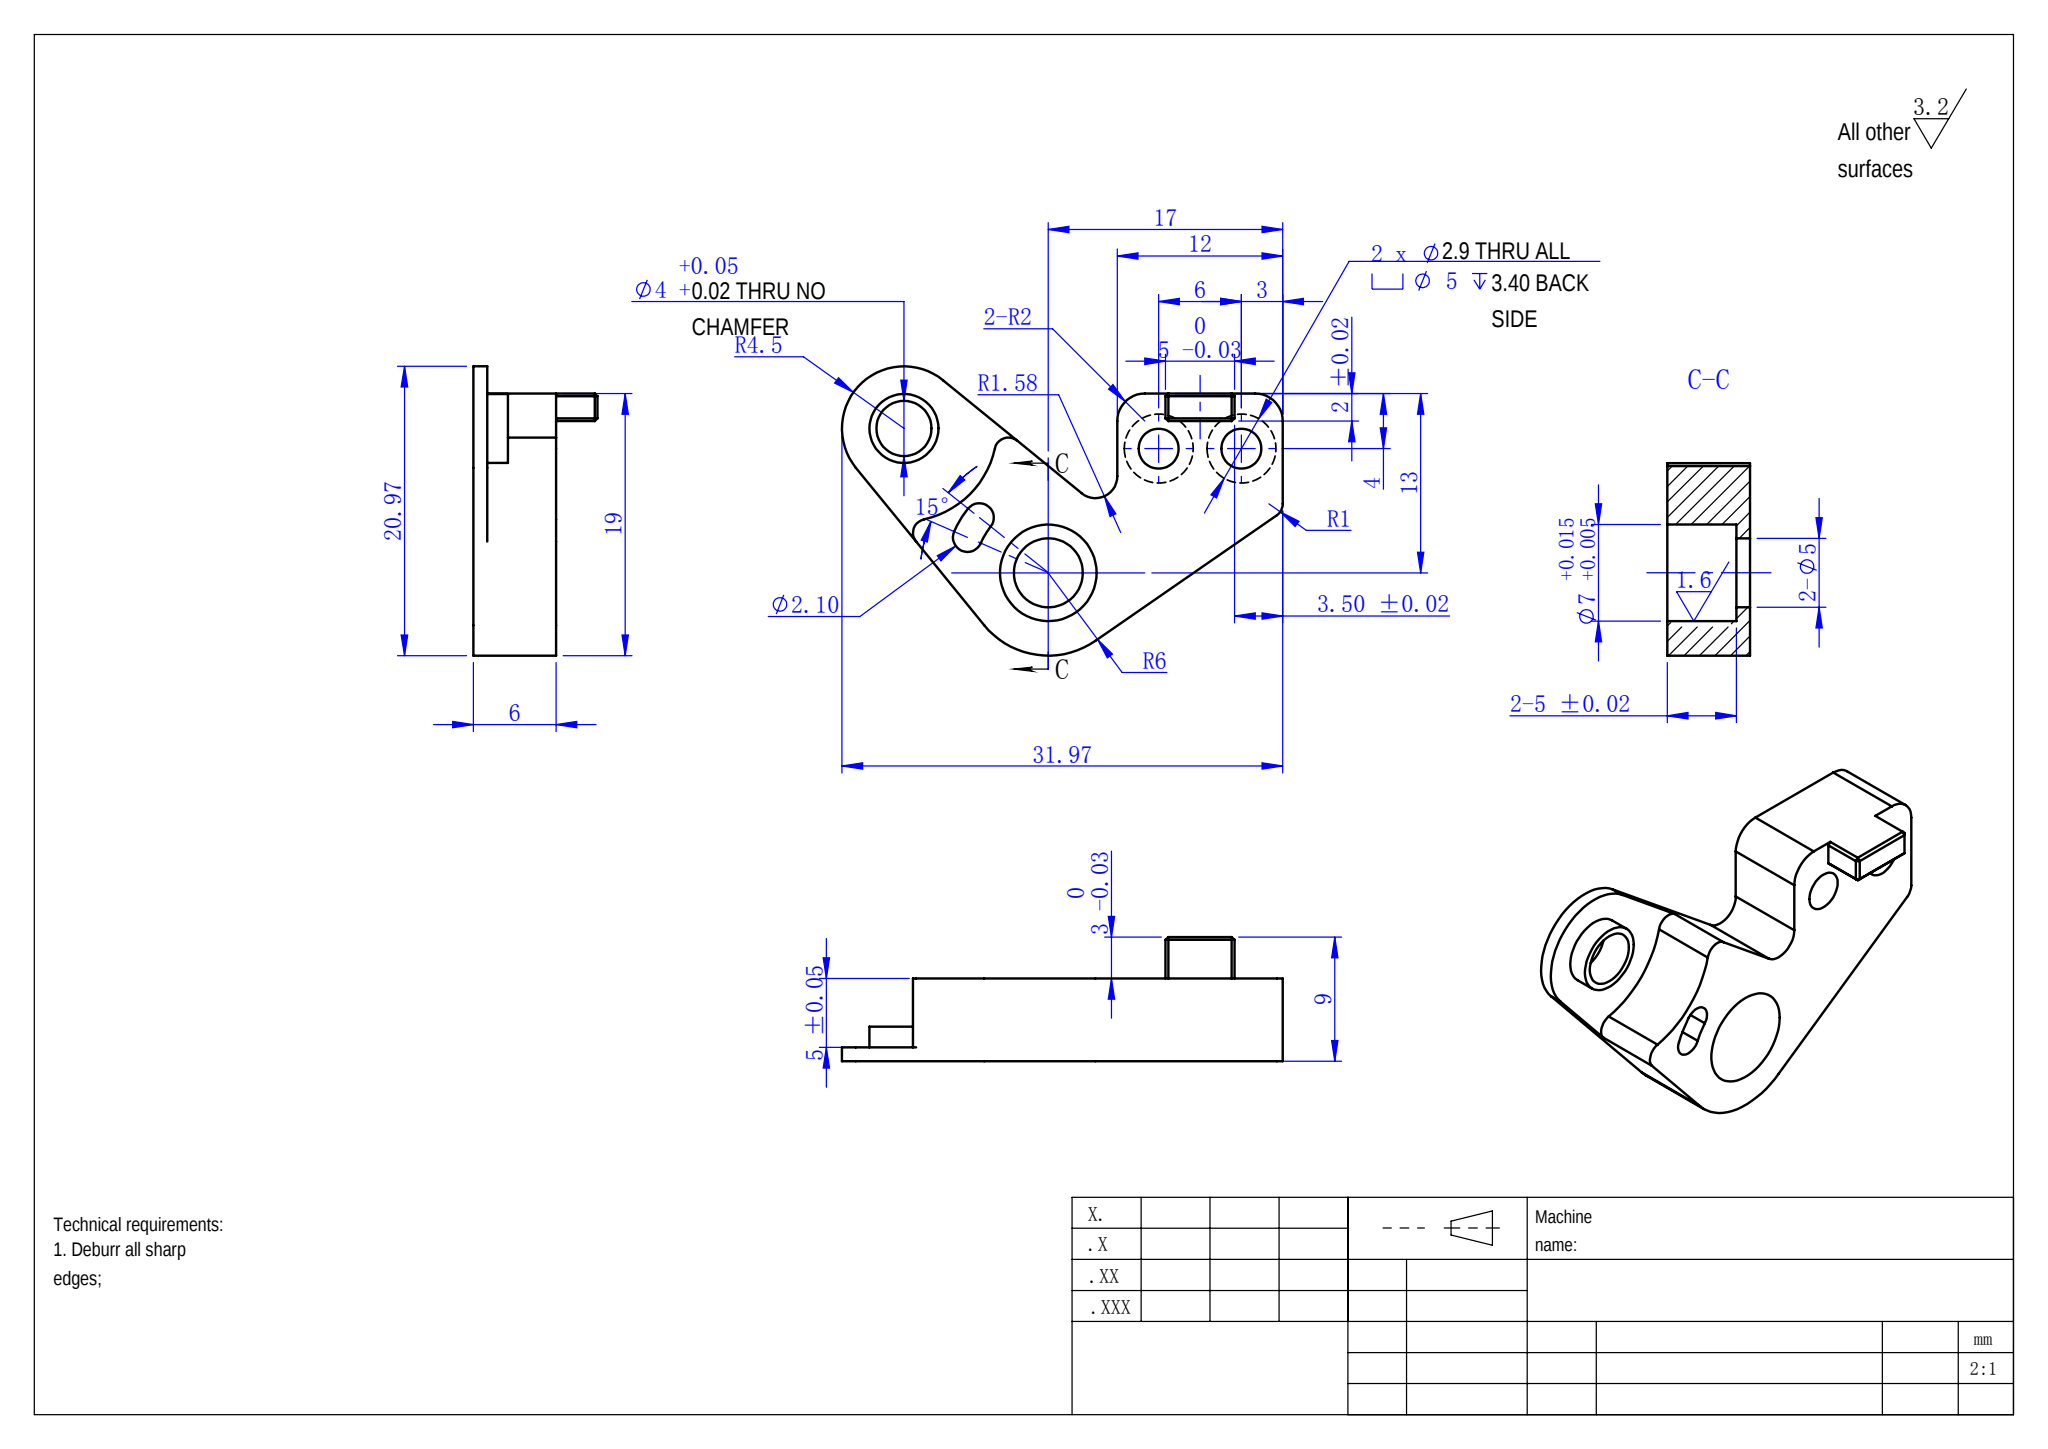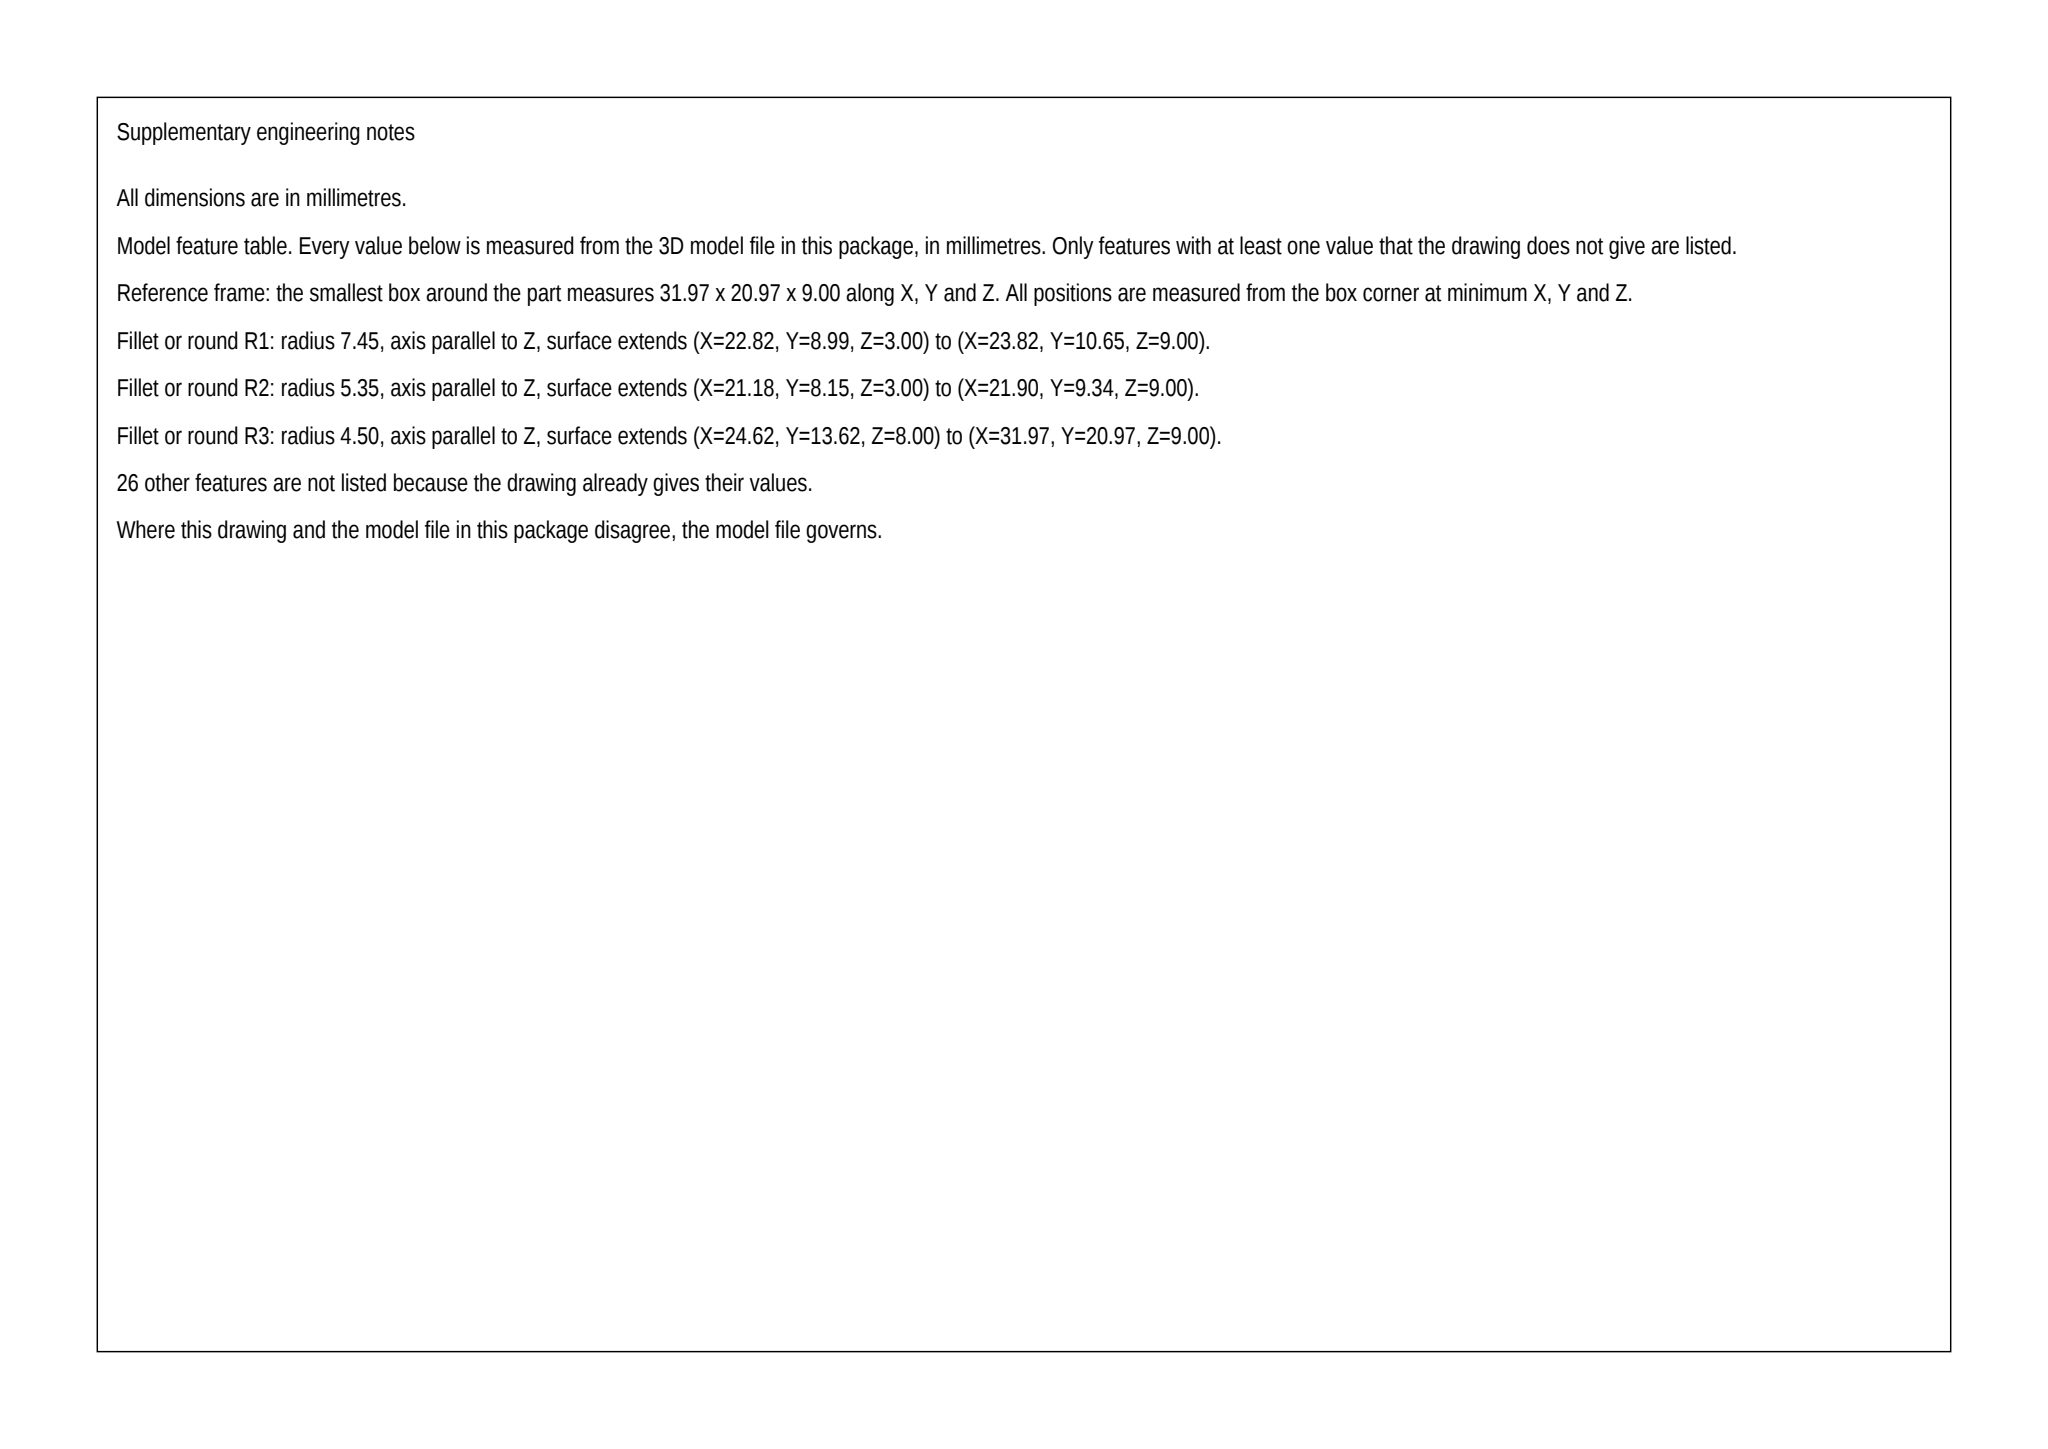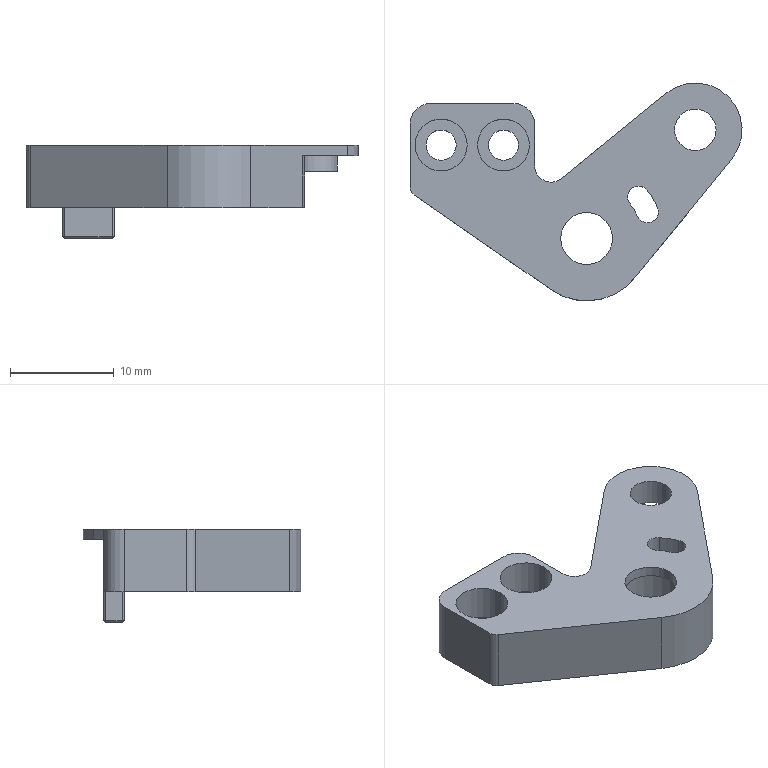Part | SolidWorks | mm | 1 solid | 59 faces | box 31.97 x 20.97 x 9 mm | volume 1507 mm3 | cylinder 30 | plane 29 | commonest cylinder face diameters 5 x8 2.9 x4 4 x4 2.1 x3 2 x3 7 x2 3.168 x1 12 x1
Drawing notes:
R1.58 notch radius centre located at X13.58/Y13.00 from the lower-left corner. | from the solid: cylinder dia 3.168 (=R1.584), axis z, pos (13.58,13.0), length 6.0
R1 half-round notch on right-hand edge: centre at X25.81/Y8.89 from the lower-left corner, 5 deep; second R1 notch centre at X19.89/Y14.81. | from the solid: cylinders dia 2.0, axis z, pos (25.81,8.89) and (19.89,14.81), length 5.0
Ø7 +0.015/+0.005 bore / R6 boss centre located at X17.00/Y6.00 from the lower-left corner. | from the solid: cylinders dia 7.0, 10.7, 12.0, 14.9, axis z, pos (17.0,6.0)
2X Ø2.9 DP 2.6 FROM NEAR FACE, CBORE Ø5 DP 3.4 FROM FAR SIDE (THRU 6 PLATE); CENTRES X3.0 Y15.0 AND X9.0 Y15.0 FROM LOWER-LEFT CORNER DATUM | from the solid: cylinders dia 2.9 len 2.6 and dia 5.0 len 3.4, both axis z at [3.0,15.0] and [9.0,15.0]
COUNTERBORED HOLE ON UPPER ARM: Ø4 DP 2.5 (Z6.5 TO Z9.0), CBORE Ø5 DP 1.5 (Z6.5 TO Z8.0), BOSS Ø9 DP 1.0 (Z8.0 TO Z9.0) ON Ø13.5; CENTRE X27.5 Y16.5 FROM LOWER-LEFT CORNER DATUM | from the solid: hole/bore Ø4 z @ [27.5,16.5] from 6.5 to 9.0; boss/shaft Ø5 @ [27.5,16.5] from 6.5 to 8.0; convex arc Ø9 @ [27.5,16.5] from 8.0 to 9.0; concave arc Ø13.5 @ [27.5,16.5] from 3.0 to 8.0
BOSS / STEP FACE LEVELS FROM BOTTOM FACE Z0: Z=5.6 AND Z=6.5 (STEP FACE Z=3.0, TOP FACES Z=8.0 AND Z=9.0 OVERALL) | from the solid: axis_planes normal z at offsets 0.0, 3.0, 5.6, 6.5, 8.0, 9.0
"Ø THROUGH, NO CHAMFER" LEADER APPLIES TO THE Ø4 HOLE ON THE UPPER ARM, CENTRE X27.5 Y16.5 FROM LOWER-LEFT CORNER DATUM: Ø4 THRU THE 2.5 THICK ARM (Z6.5 TO Z9.0 FROM BOTTOM FACE Z0), NO CHAMFER. | from the solid: cylinders: hole/bore dia 4.0, axis z at [27.5, 16.5], from 6.5 to 9.0, 360°; axis_planes z=6.5 extent x[25.0,30.0] y[14.0,19.0] (arm underside) and z=9.0 top face
ALL EDGES OF THE 5 X 2 X 3 BOTTOM TAB (TAB X3.5-8.5, Y17.0-19.0, Z0-3.0 BELOW BOTTOM FACE): CHAMFER 0.2 X 45°. | from the solid: inclined_planes at 45° with 0.2 size around tab: bbox_from [3.5,17.0,0.2], [3.5,18.8,0.2], [8.3,17.0,0.2], [8.3,18.8,0.2] size [0.2,0.2,2.8]; [3.7,17.0,0.0] and [3.7,18.8,0.0] size [4.6,0.2,0.2]; [3.5,17.2,0.0] and [8.3,17.2,0.0] size [0.2,1.6,0.2]
LOWER-LEFT INCLINED PROFILE FACE: 34.7° TO THE X AXIS (55.3° TO Y), FACE STARTS AT X0.4 Y1.1 AND RUNS 13.2 X 9.1, FULL HEIGHT Z3.0 TO Z9.0 | from the solid: inclined_planes: angle_to_xyz_axes [55.3,34.7,90.0], bbox_from [0.4,1.1,3.0], size [13.2,9.1,6.0]
UPPER INCLINED PROFILE FACE: 39.2° TO THE Y AXIS (50.8° TO X), FACE STARTS AT X14.6 Y11.8 AND RUNS 10.0 X 8.2, FULL HEIGHT Z3.0 TO Z9.0 | from the solid: inclined_planes: angle_to_xyz_axes [50.8,39.2,90.0], bbox_from [14.6,11.8,3.0], size [10.0,8.2,6.0]
STEPPED BORE AT X17.0 Y6.0 FROM LOWER-LEFT CORNER DATUM: Ø7 +0.015/+0.005 DP 5.0 FROM BOTTOM FACE Z3.0 UP TO Z8.0; Ø5 CBORE DP 1.0 FROM TOP FACE Z9.0 DOWN TO Z8.0 | from the solid: cylinders: hole/bore dia 7.0 axis z at [17.0,6.0] from 3.0 to 8.0; hole/bore dia 5.0 axis z at [17.0,6.0] from 8.0 to 9.0
PROFILE BLEND AT R6 BOSS: R5.35 CONVEX ARC 15° AND R7.45 CONCAVE ARC 15°, BOTH CENTRED X17.0 Y6.0 FROM LOWER-LEFT CORNER DATUM, FULL 6 THICK (Z3.0 TO Z9.0) | from the solid: cylinders: convex arc dia 10.7 axis z at [17.0,6.0] z3.0-9.0 arc 15°; concave arc dia 14.9 axis z at [17.0,6.0] z3.0-9.0 arc 15°
RIGHT-HAND INCLINED PROFILE FACE AT 39.2° TO X AXIS (50.8° TO Y); FACE BEGINS X21.7 Y2.2 FROM LOWER-LEFT CORNER DATUM, RUNS 9.3 X 11.4, FULL HEIGHT Z3.0 TO Z9.0 | from the solid: inclined_planes: angle_to_xyz_axes [39.2,50.8,90.0], bbox_from [21.7,2.2,3.0], size [9.3,11.4,6.0]
TOP STEP: FACE Z8.0 (1.0 BELOW TOP FACE Z9.0) COVERS THE RIGHT-HAND PORTION X19.3 TO 32.0, Y8.3 TO 21.0 FROM LOWER-LEFT CORNER DATUM; STEP BOUNDARY ON THE BOSS SIDE IS THE R4.5 (Ø9) ARC CENTRED X27.5 Y16.5, Z8.0 TO Z9.0. | from the solid: axis_planes z=8.0 extent x[19.3,32.0] y[8.3,21.0] area 72; convex arc dia 9.0 axis z at (27.5,16.5) from 8.0 to 9.0, 168 deg; axis_plane z=9.0 extent x[0,32] y[0,21]
OBROUND SLOT 2X Ø2.1 THRU Z3.0 TO Z9.0: END-HOLE CENTRES X22.0 Y10.0 AND X22.9 Y8.6 FROM LOWER-LEFT CORNER DATUM. | from the solid: concave arcs dia 2.1 axis z at (22.0,10.0) and (22.9,8.6), from 3.0 to 9.0, 180 deg each
build123d program:
from build123d import *
from build123d.topology import SkipClean

# Parameters (mm, degrees)
SKETCH1_R                                            = 2.5
SKETCH1_R_2                                          = 2
BOSS_EXTRUDE1_DEPTH                                  = 6
SKETCH2_R                                            = 3.5
CUT_EXTRUDE1_DEPTH                                   = 5
FILLET1_R                                            = 2
HOLE_SIZE_ACCORDING_TO_THE_TYPE_OF_HEXAG_D           = 2.9
HOLE_SIZE_ACCORDING_TO_THE_TYPE_OF_HEXAG_CBORE_D     = 5
HOLE_SIZE_ACCORDING_TO_THE_TYPE_OF_HEXAG_CBORE_DEPTH = 3.4
F_2_0_2_DIAMETER_HOLE1_D                             = 2
F_2_0_2_DIAMETER_HOLE1_DEPTH                         = 10
F_2_0_2_DIAMETER_HOLE1_TIP                           = 0.6009
CUT_EXTRUDE2_DEPTH                                   = 10
SKETCH12_R                                           = 3.5
CUT_EXTRUDE3_DEPTH                                   = 5
SKETCH13_R                                           = 6.75
CUT_EXTRUDE4_DEPTH                                   = 5
FILLET2_R                                            = 1
SKETCH14_W                                           = 5
SKETCH14_H                                           = 2
BOSS_EXTRUDE2_DEPTH                                  = 3
CHAMFER1_SIZE                                        = 0.2
BOSS_EXTRUDE3_START                                  = 1.5
SKETCH15_R                                           = 2.5
SKETCH15_R_2                                         = 2
BOSS_EXTRUDE3_DEPTH                                  = 1.5


with BuildPart() as part:
    # Sketch1 → Boss-Extrude1 (new body)
    with BuildSketch(Plane.XY):
        with BuildLine():
            Line((30.953, -5.378), (21.651, -16.791))
            ThreePointArc((21.651, -16.791), (17.841, -18.941), (13.584, -17.932))
            Line((13.584, -17.932), (0.4306, -8.822))
            ThreePointArc((0.4306, -8.822), (0.1142, -8.464), (0, -8))
            Line((0, -8), (0, 0))
            Line((0, 0), (12, 0))
            Line((12, 0), (12, -6))
            ThreePointArc((12, -6), (12.904, -7.431), (14.585, -7.228))
            Line((14.585, -7.228), (24.622, 0.9533))
            ThreePointArc((24.622, 0.9533), (30.647, 0.6472), (30.953, -5.378))
        make_face()
        with Locations((17, -13)):
            Circle(SKETCH1_R, mode=Mode.SUBTRACT)
        with Locations((27.465, -2.535)):
            Circle(SKETCH1_R_2, mode=Mode.SUBTRACT)
    extrude(amount=BOSS_EXTRUDE1_DEPTH)

    # Sketch2 → Cut-Extrude1 (cut)
    with BuildSketch(Plane(origin=(0, 0, 0), x_dir=(-1, 0, 0), z_dir=(0, 0, -1))):
        with Locations((-17, -13)):
            Circle(SKETCH2_R)
    extrude(amount=-CUT_EXTRUDE1_DEPTH, mode=Mode.SUBTRACT)

    # Fillet1
    fillet1_edges = [part.edges().sort_by_distance(p)[0] for p in [
        (0, 0, 3),
        (12, 0, 3),
    ]]
    fillet(fillet1_edges, radius=FILLET1_R)

    # Hole Size according to the type of hexag (through all)
    with Locations(Plane.XY.offset(6)):
        with Locations((3, -4), (9, -4)):
            CounterBoreHole(HOLE_SIZE_ACCORDING_TO_THE_TYPE_OF_HEXAG_D / 2, HOLE_SIZE_ACCORDING_TO_THE_TYPE_OF_HEXAG_CBORE_D / 2, HOLE_SIZE_ACCORDING_TO_THE_TYPE_OF_HEXAG_CBORE_DEPTH)

    # 2.0 _2_ Diameter Hole1
    with Locations(Plane.XY.offset(6)):
        with Locations((21.998, -9.003)):
            Hole(F_2_0_2_DIAMETER_HOLE1_D / 2, depth=F_2_0_2_DIAMETER_HOLE1_DEPTH)
            with Locations((0, 0, -(F_2_0_2_DIAMETER_HOLE1_DEPTH + F_2_0_2_DIAMETER_HOLE1_TIP / 2))):  # 118° drill point
                Cone(0, F_2_0_2_DIAMETER_HOLE1_D / 2, F_2_0_2_DIAMETER_HOLE1_TIP, mode=Mode.SUBTRACT)

    # Sketch11 → Cut-Extrude2 (cut)
    with BuildSketch(Plane.XY.offset(6)):
        with BuildLine():
            ThreePointArc((22.818, -8.347), (21.342, -8.183), (21.178, -9.659))
            ThreePointArc((21.178, -9.659), (21.579, -10.233), (21.901, -10.854))
            ThreePointArc((21.901, -10.854), (23.284, -11.394), (23.824, -10.011))
            ThreePointArc((23.824, -10.011), (23.376, -9.146), (22.818, -8.347))
        make_face()
    extrude(amount=-CUT_EXTRUDE2_DEPTH, mode=Mode.SUBTRACT)

    # Sketch12 → Cut-Extrude3 (cut)
    with BuildSketch(Plane(origin=(0, 0, 0), x_dir=(-1, 0, 0), z_dir=(0, 0, -1))):
        with Locations((-27.465, -2.535)):
            Circle(SKETCH12_R)
    extrude(amount=-CUT_EXTRUDE3_DEPTH, mode=Mode.SUBTRACT)

    # Sketch13 → Cut-Extrude4 (cut)
    with BuildSketch(Plane(origin=(0, 0, 0), x_dir=(-1, 0, 0), z_dir=(0, 0, -1))):
        with Locations((-27.465, -2.535)):
            Circle(SKETCH13_R)
    extrude(amount=-CUT_EXTRUDE4_DEPTH, mode=Mode.SUBTRACT)

    # Fillet2
    fillet2_edges = [part.edges().sort_by_distance(p)[0] for p in [
        (20.722, -2.225, 2.5),
        (27.775, -9.278, 2.5),
    ]]
    fillet(fillet2_edges, radius=FILLET2_R)

    # Sketch14 → Boss-Extrude2 (add)
    with BuildSketch(Plane(origin=(0, 0, 0), x_dir=(-1, 0, 0), z_dir=(0, 0, -1))):
        with Locations((-6, -1)):
            Rectangle(SKETCH14_W, SKETCH14_H)
    extrude(amount=BOSS_EXTRUDE2_DEPTH)

    # Chamfer1
    chamfer1_edges = [part.edges().sort_by_distance(p)[0] for p in [
        (3.5, -1, -3),
        (3.5, -2, -1.5),
        (6, -2, -3),
        (8.5, -2, -1.5),
        (8.5, -1, -3),
        (8.5, 0, -1.5),
        (6, 0, -3),
        (3.5, 0, -1.5),
    ]]
    chamfer(chamfer1_edges, length=CHAMFER1_SIZE)

    # Sketch15 → Boss-Extrude3 (add)
    with SkipClean():  # the faces are left unmerged after this step: merging them gives an invalid solid
        with BuildSketch(Plane(origin=(0, 0, 5), x_dir=(-1, 0, 0), z_dir=(0, 0, -1)).offset(BOSS_EXTRUDE3_START)):
            with Locations((-27.465, -2.535)):
                Circle(SKETCH15_R)
            with Locations((-27.465, -2.535)):
                Circle(SKETCH15_R_2, mode=Mode.SUBTRACT)
        extrude(amount=-BOSS_EXTRUDE3_DEPTH)


solid = part.part